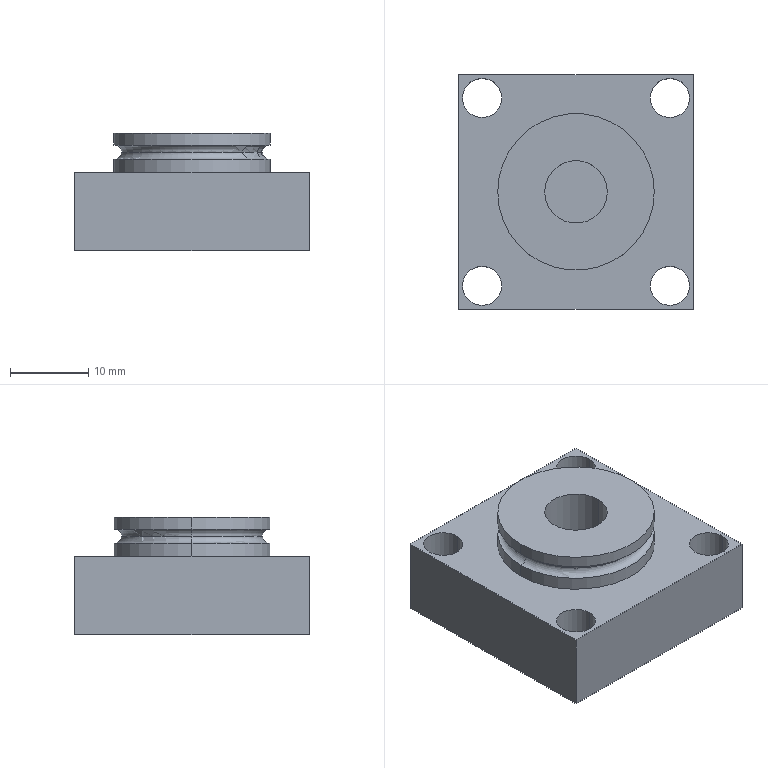Component | SolidWorks | RearEndCapAssembly-1_CylinderRearCover3-1 | 1 solid | 26 faces | box 30 x 30 x 15 mm | volume 9195 mm3 | cylinder 14 | plane 8 | torus 4 | commonest cylinder face diameters 5 x8 20 x4 8 x2
build123d program:
from build123d import *

# Parameters (mm, degrees)
SKETCH1_W         = 30
SKETCH1_H         = 30
EXTRUDE1_DEPTH    = 10
SKETCH2_R         = 10
EXTRUDE2_DEPTH    = 5
SKETCH3_R         = 4
EXTRUDE3_DEPTH    = 10
SKETCH4_R         = 2.5
EXTRUDE4_DEPTH    = 40.125
CIRPATTERN1_COUNT = 4
SKETCH5_R         = 0.9


with BuildPart() as part:
    # Sketch1 → Extrude1 (new body)
    with BuildSketch(Plane.XY):
        with Locations((-19.151, -1.261)):
            Rectangle(SKETCH1_W, SKETCH1_H)
    extrude(amount=EXTRUDE1_DEPTH)

    # Sketch2 → Extrude2 (add)
    with BuildSketch(Plane.XY.offset(10)):
        with Locations((-19.151, -1.261)):
            Circle(SKETCH2_R)
    extrude(amount=EXTRUDE2_DEPTH)

    # Sketch3 → Extrude3 (cut)
    with BuildSketch(Plane.XY.offset(15)):
        with Locations((-19.151, -1.261)):
            Circle(SKETCH3_R)
    extrude(amount=-EXTRUDE3_DEPTH, mode=Mode.SUBTRACT)

    # Sketch4 → Extrude4 (cut, through all)
    with BuildSketch(Plane.XY.offset(10)):
        with Locations((-31.151, 10.739)):
            Circle(SKETCH4_R)
    extrude4 = extrude(amount=-EXTRUDE4_DEPTH, mode=Mode.SUBTRACT)

    # CirPattern1: Extrude4 ×4 about axis
    cirpattern1_axis = Axis((-19.151, -1.261, 0), (0, 0, 1))
    for i in range(1, CIRPATTERN1_COUNT):
        add(extrude4.rotate(cirpattern1_axis, i * 360 / CIRPATTERN1_COUNT), mode=Mode.SUBTRACT)

    # Sketch5 → Cut-Revolve1 (revolve, cut)
    with BuildSketch(Plane(origin=(-19.151, 0, 0), x_dir=(0, 0, -1), z_dir=(1, 0, 0)), mode=Mode.PRIVATE) as cut_revolve1_sk:
        with Locations((-12.6, 8.639)):
            Circle(SKETCH5_R)
    revolve(cut_revolve1_sk.sketch.rotate(Axis((-19.151, -1.261, 5), (0, 0, 1)), 90), axis=Axis((-19.151, -1.261, 5), (0, 0, 1)), mode=Mode.SUBTRACT)


solid = part.part

# Placed as in the assembly
solid = solid.moved(Location((25.276, -0.3856, -7.5), (0, 0, 0)))
STEP:
#1=CARTESIAN_POINT('',(-0.1526,-0.06482,0.1656));
#2=VERTEX_POINT('',#1);
#3=CARTESIAN_POINT('',(-0.1132,-0.06482,0.2008));
#4=VERTEX_POINT('',#3);
#5=CARTESIAN_POINT('',(-0.1486,-0.06482,0.2008));
#6=DIRECTION('',(0.,-1.,0.));
#7=DIRECTION('',(0.,0.,-1.));
#8=AXIS2_PLACEMENT_3D('',#5,#6,#7);
#9=CIRCLE('',#8,0.03543);
#10=EDGE_CURVE('',#2,#4,#9,.T.);
#11=ORIENTED_EDGE('',*,*,#10,.T.);
#12=CARTESIAN_POINT('',(0.5955,-0.06482,0.2008));
#13=VERTEX_POINT('',#12);
#14=CARTESIAN_POINT('',(0.2411,-0.06482,0.2008));
#15=DIRECTION('',(0.,0.,-1.));
#16=DIRECTION('',(-1.,0.,0.));
#17=AXIS2_PLACEMENT_3D('',#14,#15,#16);
#18=CIRCLE('',#17,0.3543);
#19=EDGE_CURVE('',#4,#13,#18,.T.);
#20=ORIENTED_EDGE('',*,*,#19,.T.);
#21=CARTESIAN_POINT('',(0.6348,-0.06482,0.1656));
#22=VERTEX_POINT('',#21);
#23=CARTESIAN_POINT('',(0.6309,-0.06482,0.2008));
#24=DIRECTION('',(-0.,1.,0.));
#25=DIRECTION('',(-1.,-0.,0.));
#26=AXIS2_PLACEMENT_3D('',#23,#24,#25);
#27=CIRCLE('',#26,0.03543);
#28=EDGE_CURVE('',#22,#13,#27,.T.);
#29=ORIENTED_EDGE('',*,*,#28,.F.);
#30=CARTESIAN_POINT('',(0.2411,-0.06482,0.1656));
#31=DIRECTION('',(0.,0.,-1.));
#32=DIRECTION('',(1.,0.,0.));
#33=AXIS2_PLACEMENT_3D('',#30,#31,#32);
#34=CIRCLE('',#33,0.3937);
#35=EDGE_CURVE('',#2,#22,#34,.T.);
#36=ORIENTED_EDGE('',*,*,#35,.F.);
#37=EDGE_LOOP('',(#11,#20,#29,#36));
#38=FACE_OUTER_BOUND('',#37,.T.);
#39=CARTESIAN_POINT('',(0.2411,-0.06482,0.2008));
#40=DIRECTION('',(0.,0.,-1.));
#41=DIRECTION('',(-1.,0.,0.));
#42=AXIS2_PLACEMENT_3D('',#39,#40,#41);
#43=TOROIDAL_SURFACE('',#42,0.3898,0.03543);
#44=ADVANCED_FACE('',(#38),#43,.F.);
#45=ORIENTED_EDGE('',*,*,#28,.T.);
#46=CARTESIAN_POINT('',(0.2411,-0.06482,0.2008));
#47=DIRECTION('',(0.,0.,-1.));
#48=DIRECTION('',(-1.,0.,0.));
#49=AXIS2_PLACEMENT_3D('',#46,#47,#48);
#50=CIRCLE('',#49,0.3543);
#51=EDGE_CURVE('',#13,#4,#50,.T.);
#52=ORIENTED_EDGE('',*,*,#51,.T.);
#53=ORIENTED_EDGE('',*,*,#10,.F.);
#54=CARTESIAN_POINT('',(0.2411,-0.06482,0.1656));
#55=DIRECTION('',(0.,0.,-1.));
#56=DIRECTION('',(1.,0.,0.));
#57=AXIS2_PLACEMENT_3D('',#54,#55,#56);
#58=CIRCLE('',#57,0.3937);
#59=EDGE_CURVE('',#22,#2,#58,.T.);
#60=ORIENTED_EDGE('',*,*,#59,.F.);
#61=EDGE_LOOP('',(#45,#52,#53,#60));
#62=FACE_OUTER_BOUND('',#61,.T.);
#63=CARTESIAN_POINT('',(0.2411,-0.06482,0.2008));
#64=DIRECTION('',(0.,0.,-1.));
#65=DIRECTION('',(-1.,0.,0.));
#66=AXIS2_PLACEMENT_3D('',#63,#64,#65);
#67=TOROIDAL_SURFACE('',#66,0.3898,0.03543);
#68=ADVANCED_FACE('',(#62),#67,.F.);
#69=CARTESIAN_POINT('',(0.6348,-0.06482,0.2953));
#70=VERTEX_POINT('',#69);
#71=CARTESIAN_POINT('',(-0.1526,-0.06482,0.2953));
#72=VERTEX_POINT('',#71);
#73=CARTESIAN_POINT('',(0.2411,-0.06482,0.2953));
#74=DIRECTION('',(0.,0.,1.));
#75=DIRECTION('',(1.,0.,0.));
#76=AXIS2_PLACEMENT_3D('',#73,#74,#75);
#77=CIRCLE('',#76,0.3937);
#78=EDGE_CURVE('',#70,#72,#77,.T.);
#79=ORIENTED_EDGE('',*,*,#78,.F.);
#80=CARTESIAN_POINT('',(0.6348,-0.06482,0.236));
#81=VERTEX_POINT('',#80);
#82=CARTESIAN_POINT('',(0.6348,-0.06482,0.2953));
#83=DIRECTION('',(0.,0.,-1.));
#84=VECTOR('',#83,39.37);
#85=LINE('',#82,#84);
#86=EDGE_CURVE('',#70,#81,#85,.T.);
#87=ORIENTED_EDGE('',*,*,#86,.T.);
#88=CARTESIAN_POINT('',(-0.1526,-0.06482,0.236));
#89=VERTEX_POINT('',#88);
#90=CARTESIAN_POINT('',(0.2411,-0.06482,0.236));
#91=DIRECTION('',(0.,0.,1.));
#92=DIRECTION('',(-1.,0.,0.));
#93=AXIS2_PLACEMENT_3D('',#90,#91,#92);
#94=CIRCLE('',#93,0.3937);
#95=EDGE_CURVE('',#81,#89,#94,.T.);
#96=ORIENTED_EDGE('',*,*,#95,.T.);
#97=CARTESIAN_POINT('',(-0.1526,-0.06482,0.2953));
#98=DIRECTION('',(0.,0.,-1.));
#99=VECTOR('',#98,39.37);
#100=LINE('',#97,#99);
#101=EDGE_CURVE('',#72,#89,#100,.T.);
#102=ORIENTED_EDGE('',*,*,#101,.F.);
#103=EDGE_LOOP('',(#79,#87,#96,#102));
#104=FACE_OUTER_BOUND('',#103,.T.);
#105=CARTESIAN_POINT('',(0.2411,-0.06482,0.2953));
#106=DIRECTION('',(0.,0.,-1.));
#107=DIRECTION('',(-1.,0.,0.));
#108=AXIS2_PLACEMENT_3D('',#105,#106,#107);
#109=CYLINDRICAL_SURFACE('',#108,0.3937);
#110=ADVANCED_FACE('',(#104),#109,.T.);
#111=CARTESIAN_POINT('',(0.08366,-0.06482,-0.09843));
#112=VERTEX_POINT('',#111);
#113=CARTESIAN_POINT('',(0.3986,-0.06482,-0.09843));
#114=VERTEX_POINT('',#113);
#115=CARTESIAN_POINT('',(0.2411,-0.06482,-0.09843));
#116=DIRECTION('',(0.,0.,1.));
#117=DIRECTION('',(1.,0.,0.));
#118=AXIS2_PLACEMENT_3D('',#115,#116,#117);
#119=CIRCLE('',#118,0.1575);
#120=EDGE_CURVE('',#112,#114,#119,.T.);
#121=ORIENTED_EDGE('',*,*,#120,.F.);
#122=CARTESIAN_POINT('',(0.08366,-0.06482,0.2953));
#123=VERTEX_POINT('',#122);
#124=CARTESIAN_POINT('',(0.08366,-0.06482,-0.09843));
#125=DIRECTION('',(0.,0.,1.));
#126=VECTOR('',#125,39.37);
#127=LINE('',#124,#126);
#128=EDGE_CURVE('',#112,#123,#127,.T.);
#129=ORIENTED_EDGE('',*,*,#128,.T.);
#130=CARTESIAN_POINT('',(0.3986,-0.06482,0.2953));
#131=VERTEX_POINT('',#130);
#132=CARTESIAN_POINT('',(0.2411,-0.06482,0.2953));
#133=DIRECTION('',(0.,0.,1.));
#134=DIRECTION('',(1.,0.,0.));
#135=AXIS2_PLACEMENT_3D('',#132,#133,#134);
#136=CIRCLE('',#135,0.1575);
#137=EDGE_CURVE('',#123,#131,#136,.T.);
#138=ORIENTED_EDGE('',*,*,#137,.T.);
#139=CARTESIAN_POINT('',(0.3986,-0.06482,-0.09843));
#140=DIRECTION('',(0.,0.,1.));
#141=VECTOR('',#140,39.37);
#142=LINE('',#139,#141);
#143=EDGE_CURVE('',#114,#131,#142,.T.);
#144=ORIENTED_EDGE('',*,*,#143,.F.);
#145=EDGE_LOOP('',(#121,#129,#138,#144));
#146=FACE_OUTER_BOUND('',#145,.T.);
#147=CARTESIAN_POINT('',(0.2411,-0.06482,-0.09843));
#148=DIRECTION('',(0.,0.,1.));
#149=DIRECTION('',(1.,0.,0.));
#150=AXIS2_PLACEMENT_3D('',#147,#148,#149);
#151=CYLINDRICAL_SURFACE('',#150,0.1575);
#152=ADVANCED_FACE('',(#146),#151,.F.);
#153=ORIENTED_EDGE('',*,*,#51,.F.);
#154=CARTESIAN_POINT('',(0.6309,-0.06482,0.2008));
#155=DIRECTION('',(-0.,1.,0.));
#156=DIRECTION('',(-1.,-0.,0.));
#157=AXIS2_PLACEMENT_3D('',#154,#155,#156);
#158=CIRCLE('',#157,0.03543);
#159=EDGE_CURVE('',#13,#81,#158,.T.);
#160=ORIENTED_EDGE('',*,*,#159,.T.);
#161=CARTESIAN_POINT('',(0.2411,-0.06482,0.236));
#162=DIRECTION('',(0.,0.,1.));
#163=DIRECTION('',(-1.,0.,0.));
#164=AXIS2_PLACEMENT_3D('',#161,#162,#163);
#165=CIRCLE('',#164,0.3937);
#166=EDGE_CURVE('',#89,#81,#165,.T.);
#167=ORIENTED_EDGE('',*,*,#166,.F.);
#168=CARTESIAN_POINT('',(-0.1486,-0.06482,0.2008));
#169=DIRECTION('',(0.,-1.,0.));
#170=DIRECTION('',(0.,0.,-1.));
#171=AXIS2_PLACEMENT_3D('',#168,#169,#170);
#172=CIRCLE('',#171,0.03543);
#173=EDGE_CURVE('',#4,#89,#172,.T.);
#174=ORIENTED_EDGE('',*,*,#173,.F.);
#175=EDGE_LOOP('',(#153,#160,#167,#174));
#176=FACE_OUTER_BOUND('',#175,.T.);
#177=CARTESIAN_POINT('',(0.2411,-0.06482,0.2008));
#178=DIRECTION('',(0.,0.,-1.));
#179=DIRECTION('',(-1.,0.,0.));
#180=AXIS2_PLACEMENT_3D('',#177,#178,#179);
#181=TOROIDAL_SURFACE('',#180,0.3898,0.03543);
#182=ADVANCED_FACE('',(#176),#181,.F.);
#183=CARTESIAN_POINT('',(0.6152,0.4076,-0.2953));
#184=VERTEX_POINT('',#183);
#185=CARTESIAN_POINT('',(0.812,0.4076,-0.2953));
#186=VERTEX_POINT('',#185);
#187=CARTESIAN_POINT('',(0.7136,0.4076,-0.2953));
#188=DIRECTION('',(0.,0.,1.));
#189=DIRECTION('',(0.,-1.,0.));
#190=AXIS2_PLACEMENT_3D('',#187,#188,#189);
#191=CIRCLE('',#190,0.09843);
#192=EDGE_CURVE('',#184,#186,#191,.T.);
#193=ORIENTED_EDGE('',*,*,#192,.F.);
#194=CARTESIAN_POINT('',(0.6152,0.4076,0.09843));
#195=VERTEX_POINT('',#194);
#196=CARTESIAN_POINT('',(0.6152,0.4076,-0.2953));
#197=DIRECTION('',(0.,0.,1.));
#198=VECTOR('',#197,39.37);
#199=LINE('',#196,#198);
#200=EDGE_CURVE('',#184,#195,#199,.T.);
#201=ORIENTED_EDGE('',*,*,#200,.T.);
#202=CARTESIAN_POINT('',(0.812,0.4076,0.09843));
#203=VERTEX_POINT('',#202);
#204=CARTESIAN_POINT('',(0.7136,0.4076,0.09843));
#205=DIRECTION('',(0.,0.,1.));
#206=DIRECTION('',(0.,-1.,0.));
#207=AXIS2_PLACEMENT_3D('',#204,#205,#206);
#208=CIRCLE('',#207,0.09843);
#209=EDGE_CURVE('',#195,#203,#208,.T.);
#210=ORIENTED_EDGE('',*,*,#209,.T.);
#211=CARTESIAN_POINT('',(0.812,0.4076,-0.2953));
#212=DIRECTION('',(0.,0.,1.));
#213=VECTOR('',#212,39.37);
#214=LINE('',#211,#213);
#215=EDGE_CURVE('',#186,#203,#214,.T.);
#216=ORIENTED_EDGE('',*,*,#215,.F.);
#217=EDGE_LOOP('',(#193,#201,#210,#216));
#218=FACE_OUTER_BOUND('',#217,.T.);
#219=CARTESIAN_POINT('',(0.7136,0.4076,-0.2953));
#220=DIRECTION('',(0.,0.,1.));
#221=DIRECTION('',(1.,0.,0.));
#222=AXIS2_PLACEMENT_3D('',#219,#220,#221);
#223=CYLINDRICAL_SURFACE('',#222,0.09843);
#224=ADVANCED_FACE('',(#218),#223,.F.);
#225=CARTESIAN_POINT('',(0.6152,-0.5373,-0.2953));
#226=VERTEX_POINT('',#225);
#227=CARTESIAN_POINT('',(0.812,-0.5373,-0.2953));
#228=VERTEX_POINT('',#227);
#229=CARTESIAN_POINT('',(0.7136,-0.5373,-0.2953));
#230=DIRECTION('',(0.,0.,1.));
#231=DIRECTION('',(-1.,-0.,0.));
#232=AXIS2_PLACEMENT_3D('',#229,#230,#231);
#233=CIRCLE('',#232,0.09843);
#234=EDGE_CURVE('',#226,#228,#233,.T.);
#235=ORIENTED_EDGE('',*,*,#234,.F.);
#236=CARTESIAN_POINT('',(0.6152,-0.5373,0.09843));
#237=VERTEX_POINT('',#236);
#238=CARTESIAN_POINT('',(0.6152,-0.5373,-0.2953));
#239=DIRECTION('',(0.,0.,1.));
#240=VECTOR('',#239,39.37);
#241=LINE('',#238,#240);
#242=EDGE_CURVE('',#226,#237,#241,.T.);
#243=ORIENTED_EDGE('',*,*,#242,.T.);
#244=CARTESIAN_POINT('',(0.812,-0.5373,0.09843));
#245=VERTEX_POINT('',#244);
#246=CARTESIAN_POINT('',(0.7136,-0.5373,0.09843));
#247=DIRECTION('',(0.,0.,1.));
#248=DIRECTION('',(-1.,-0.,0.));
#249=AXIS2_PLACEMENT_3D('',#246,#247,#248);
#250=CIRCLE('',#249,0.09843);
#251=EDGE_CURVE('',#237,#245,#250,.T.);
#252=ORIENTED_EDGE('',*,*,#251,.T.);
#253=CARTESIAN_POINT('',(0.812,-0.5373,-0.2953));
#254=DIRECTION('',(0.,0.,1.));
#255=VECTOR('',#254,39.37);
#256=LINE('',#253,#255);
#257=EDGE_CURVE('',#228,#245,#256,.T.);
#258=ORIENTED_EDGE('',*,*,#257,.F.);
#259=EDGE_LOOP('',(#235,#243,#252,#258));
#260=FACE_OUTER_BOUND('',#259,.T.);
#261=CARTESIAN_POINT('',(0.7136,-0.5373,-0.2953));
#262=DIRECTION('',(0.,0.,1.));
#263=DIRECTION('',(1.,0.,0.));
#264=AXIS2_PLACEMENT_3D('',#261,#262,#263);
#265=CYLINDRICAL_SURFACE('',#264,0.09843);
#266=ADVANCED_FACE('',(#260),#265,.F.);
#267=CARTESIAN_POINT('',(-0.3297,-0.5373,-0.2953));
#268=VERTEX_POINT('',#267);
#269=CARTESIAN_POINT('',(-0.1329,-0.5373,-0.2953));
#270=VERTEX_POINT('',#269);
#271=CARTESIAN_POINT('',(-0.2313,-0.5373,-0.2953));
#272=DIRECTION('',(0.,0.,1.));
#273=DIRECTION('',(-0.,1.,0.));
#274=AXIS2_PLACEMENT_3D('',#271,#272,#273);
#275=CIRCLE('',#274,0.09843);
#276=EDGE_CURVE('',#268,#270,#275,.T.);
#277=ORIENTED_EDGE('',*,*,#276,.F.);
#278=CARTESIAN_POINT('',(-0.3297,-0.5373,0.09843));
#279=VERTEX_POINT('',#278);
#280=CARTESIAN_POINT('',(-0.3297,-0.5373,-0.2953));
#281=DIRECTION('',(0.,0.,1.));
#282=VECTOR('',#281,39.37);
#283=LINE('',#280,#282);
#284=EDGE_CURVE('',#268,#279,#283,.T.);
#285=ORIENTED_EDGE('',*,*,#284,.T.);
#286=CARTESIAN_POINT('',(-0.1329,-0.5373,0.09843));
#287=VERTEX_POINT('',#286);
#288=CARTESIAN_POINT('',(-0.2313,-0.5373,0.09843));
#289=DIRECTION('',(0.,0.,1.));
#290=DIRECTION('',(-0.,1.,0.));
#291=AXIS2_PLACEMENT_3D('',#288,#289,#290);
#292=CIRCLE('',#291,0.09843);
#293=EDGE_CURVE('',#279,#287,#292,.T.);
#294=ORIENTED_EDGE('',*,*,#293,.T.);
#295=CARTESIAN_POINT('',(-0.1329,-0.5373,-0.2953));
#296=DIRECTION('',(0.,0.,1.));
#297=VECTOR('',#296,39.37);
#298=LINE('',#295,#297);
#299=EDGE_CURVE('',#270,#287,#298,.T.);
#300=ORIENTED_EDGE('',*,*,#299,.F.);
#301=EDGE_LOOP('',(#277,#285,#294,#300));
#302=FACE_OUTER_BOUND('',#301,.T.);
#303=CARTESIAN_POINT('',(-0.2313,-0.5373,-0.2953));
#304=DIRECTION('',(0.,0.,1.));
#305=DIRECTION('',(1.,0.,0.));
#306=AXIS2_PLACEMENT_3D('',#303,#304,#305);
#307=CYLINDRICAL_SURFACE('',#306,0.09843);
#308=ADVANCED_FACE('',(#302),#307,.F.);
#309=CARTESIAN_POINT('',(-0.3297,0.4076,-0.2953));
#310=VERTEX_POINT('',#309);
#311=CARTESIAN_POINT('',(-0.1329,0.4076,-0.2953));
#312=VERTEX_POINT('',#311);
#313=CARTESIAN_POINT('',(-0.2313,0.4076,-0.2953));
#314=DIRECTION('',(0.,0.,1.));
#315=DIRECTION('',(1.,0.,0.));
#316=AXIS2_PLACEMENT_3D('',#313,#314,#315);
#317=CIRCLE('',#316,0.09843);
#318=EDGE_CURVE('',#310,#312,#317,.T.);
#319=ORIENTED_EDGE('',*,*,#318,.F.);
#320=CARTESIAN_POINT('',(-0.3297,0.4076,0.09843));
#321=VERTEX_POINT('',#320);
#322=CARTESIAN_POINT('',(-0.3297,0.4076,-0.2953));
#323=DIRECTION('',(0.,0.,1.));
#324=VECTOR('',#323,39.37);
#325=LINE('',#322,#324);
#326=EDGE_CURVE('',#310,#321,#325,.T.);
#327=ORIENTED_EDGE('',*,*,#326,.T.);
#328=CARTESIAN_POINT('',(-0.1329,0.4076,0.09843));
#329=VERTEX_POINT('',#328);
#330=CARTESIAN_POINT('',(-0.2313,0.4076,0.09843));
#331=DIRECTION('',(0.,0.,1.));
#332=DIRECTION('',(1.,0.,0.));
#333=AXIS2_PLACEMENT_3D('',#330,#331,#332);
#334=CIRCLE('',#333,0.09843);
#335=EDGE_CURVE('',#321,#329,#334,.T.);
#336=ORIENTED_EDGE('',*,*,#335,.T.);
#337=CARTESIAN_POINT('',(-0.1329,0.4076,-0.2953));
#338=DIRECTION('',(0.,0.,1.));
#339=VECTOR('',#338,39.37);
#340=LINE('',#337,#339);
#341=EDGE_CURVE('',#312,#329,#340,.T.);
#342=ORIENTED_EDGE('',*,*,#341,.F.);
#343=EDGE_LOOP('',(#319,#327,#336,#342));
#344=FACE_OUTER_BOUND('',#343,.T.);
#345=CARTESIAN_POINT('',(-0.2313,0.4076,-0.2953));
#346=DIRECTION('',(0.,0.,1.));
#347=DIRECTION('',(1.,0.,0.));
#348=AXIS2_PLACEMENT_3D('',#345,#346,#347);
#349=CYLINDRICAL_SURFACE('',#348,0.09843);
#350=ADVANCED_FACE('',(#344),#349,.F.);
#351=ORIENTED_EDGE('',*,*,#35,.T.);
#352=CARTESIAN_POINT('',(0.6348,-0.06482,0.09843));
#353=VERTEX_POINT('',#352);
#354=CARTESIAN_POINT('',(0.6348,-0.06482,0.2953));
#355=DIRECTION('',(0.,0.,-1.));
#356=VECTOR('',#355,39.37);
#357=LINE('',#354,#356);
#358=EDGE_CURVE('',#22,#353,#357,.T.);
#359=ORIENTED_EDGE('',*,*,#358,.T.);
#360=CARTESIAN_POINT('',(-0.1526,-0.06482,0.09843));
#361=VERTEX_POINT('',#360);
#362=CARTESIAN_POINT('',(0.2411,-0.06482,0.09843));
#363=DIRECTION('',(0.,0.,1.));
#364=DIRECTION('',(1.,0.,0.));
#365=AXIS2_PLACEMENT_3D('',#362,#363,#364);
#366=CIRCLE('',#365,0.3937);
#367=EDGE_CURVE('',#353,#361,#366,.T.);
#368=ORIENTED_EDGE('',*,*,#367,.T.);
#369=CARTESIAN_POINT('',(-0.1526,-0.06482,0.2953));
#370=DIRECTION('',(0.,0.,-1.));
#371=VECTOR('',#370,39.37);
#372=LINE('',#369,#371);
#373=EDGE_CURVE('',#2,#361,#372,.T.);
#374=ORIENTED_EDGE('',*,*,#373,.F.);
#375=EDGE_LOOP('',(#351,#359,#368,#374));
#376=FACE_OUTER_BOUND('',#375,.T.);
#377=CARTESIAN_POINT('',(0.2411,-0.06482,0.2953));
#378=DIRECTION('',(0.,0.,-1.));
#379=DIRECTION('',(-1.,0.,0.));
#380=AXIS2_PLACEMENT_3D('',#377,#378,#379);
#381=CYLINDRICAL_SURFACE('',#380,0.3937);
#382=ADVANCED_FACE('',(#376),#381,.T.);
#383=ORIENTED_EDGE('',*,*,#358,.F.);
#384=ORIENTED_EDGE('',*,*,#59,.T.);
#385=ORIENTED_EDGE('',*,*,#373,.T.);
#386=CARTESIAN_POINT('',(0.2411,-0.06482,0.09843));
#387=DIRECTION('',(0.,0.,1.));
#388=DIRECTION('',(1.,0.,0.));
#389=AXIS2_PLACEMENT_3D('',#386,#387,#388);
#390=CIRCLE('',#389,0.3937);
#391=EDGE_CURVE('',#361,#353,#390,.T.);
#392=ORIENTED_EDGE('',*,*,#391,.T.);
#393=EDGE_LOOP('',(#383,#384,#385,#392));
#394=FACE_OUTER_BOUND('',#393,.T.);
#395=CARTESIAN_POINT('',(0.2411,-0.06482,0.2953));
#396=DIRECTION('',(0.,0.,-1.));
#397=DIRECTION('',(-1.,0.,0.));
#398=AXIS2_PLACEMENT_3D('',#395,#396,#397);
#399=CYLINDRICAL_SURFACE('',#398,0.3937);
#400=ADVANCED_FACE('',(#394),#399,.T.);
#401=CARTESIAN_POINT('',(0.7136,0.4076,0.09843));
#402=DIRECTION('',(0.,0.,1.));
#403=DIRECTION('',(0.,-1.,0.));
#404=AXIS2_PLACEMENT_3D('',#401,#402,#403);
#405=CIRCLE('',#404,0.09843);
#406=EDGE_CURVE('',#203,#195,#405,.T.);
#407=ORIENTED_EDGE('',*,*,#406,.F.);
#408=ORIENTED_EDGE('',*,*,#209,.F.);
#409=EDGE_LOOP('',(#407,#408));
#410=FACE_BOUND('',#409,.T.);
#411=CARTESIAN_POINT('',(0.7136,-0.5373,0.09843));
#412=DIRECTION('',(0.,0.,1.));
#413=DIRECTION('',(-1.,-0.,0.));
#414=AXIS2_PLACEMENT_3D('',#411,#412,#413);
#415=CIRCLE('',#414,0.09843);
#416=EDGE_CURVE('',#245,#237,#415,.T.);
#417=ORIENTED_EDGE('',*,*,#416,.F.);
#418=ORIENTED_EDGE('',*,*,#251,.F.);
#419=EDGE_LOOP('',(#417,#418));
#420=FACE_BOUND('',#419,.T.);
#421=CARTESIAN_POINT('',(-0.2313,-0.5373,0.09843));
#422=DIRECTION('',(0.,0.,1.));
#423=DIRECTION('',(-0.,1.,0.));
#424=AXIS2_PLACEMENT_3D('',#421,#422,#423);
#425=CIRCLE('',#424,0.09843);
#426=EDGE_CURVE('',#287,#279,#425,.T.);
#427=ORIENTED_EDGE('',*,*,#426,.F.);
#428=ORIENTED_EDGE('',*,*,#293,.F.);
#429=EDGE_LOOP('',(#427,#428));
#430=FACE_BOUND('',#429,.T.);
#431=CARTESIAN_POINT('',(-0.2313,0.4076,0.09843));
#432=DIRECTION('',(0.,0.,1.));
#433=DIRECTION('',(1.,0.,0.));
#434=AXIS2_PLACEMENT_3D('',#431,#432,#433);
#435=CIRCLE('',#434,0.09843);
#436=EDGE_CURVE('',#329,#321,#435,.T.);
#437=ORIENTED_EDGE('',*,*,#436,.F.);
#438=ORIENTED_EDGE('',*,*,#335,.F.);
#439=EDGE_LOOP('',(#437,#438));
#440=FACE_BOUND('',#439,.T.);
#441=CARTESIAN_POINT('',(-0.3494,0.5257,0.09843));
#442=VERTEX_POINT('',#441);
#443=CARTESIAN_POINT('',(-0.3494,-0.6554,0.09843));
#444=VERTEX_POINT('',#443);
#445=CARTESIAN_POINT('',(-0.3494,0.5257,0.09843));
#446=DIRECTION('',(0.,-1.,0.));
#447=VECTOR('',#446,39.37);
#448=LINE('',#445,#447);
#449=EDGE_CURVE('',#442,#444,#448,.T.);
#450=ORIENTED_EDGE('',*,*,#449,.T.);
#451=CARTESIAN_POINT('',(0.8317,-0.6554,0.09843));
#452=VERTEX_POINT('',#451);
#453=CARTESIAN_POINT('',(-0.3494,-0.6554,0.09843));
#454=DIRECTION('',(1.,0.,0.));
#455=VECTOR('',#454,39.37);
#456=LINE('',#453,#455);
#457=EDGE_CURVE('',#444,#452,#456,.T.);
#458=ORIENTED_EDGE('',*,*,#457,.T.);
#459=CARTESIAN_POINT('',(0.8317,0.5257,0.09843));
#460=VERTEX_POINT('',#459);
#461=CARTESIAN_POINT('',(0.8317,0.5257,0.09843));
#462=DIRECTION('',(-0.,1.,0.));
#463=VECTOR('',#462,39.37);
#464=LINE('',#461,#463);
#465=EDGE_CURVE('',#452,#460,#464,.T.);
#466=ORIENTED_EDGE('',*,*,#465,.T.);
#467=CARTESIAN_POINT('',(-0.3494,0.5257,0.09843));
#468=DIRECTION('',(-1.,0.,0.));
#469=VECTOR('',#468,39.37);
#470=LINE('',#467,#469);
#471=EDGE_CURVE('',#460,#442,#470,.T.);
#472=ORIENTED_EDGE('',*,*,#471,.T.);
#473=EDGE_LOOP('',(#450,#458,#466,#472));
#474=FACE_OUTER_BOUND('',#473,.T.);
#475=ORIENTED_EDGE('',*,*,#391,.F.);
#476=ORIENTED_EDGE('',*,*,#367,.F.);
#477=EDGE_LOOP('',(#475,#476));
#478=FACE_BOUND('',#477,.T.);
#479=CARTESIAN_POINT('',(-0.3494,-0.6554,0.09843));
#480=DIRECTION('',(0.,0.,1.));
#481=DIRECTION('',(1.,0.,0.));
#482=AXIS2_PLACEMENT_3D('',#479,#480,#481);
#483=PLANE('',#482);
#484=ADVANCED_FACE('',(#410,#420,#430,#440,#474,#478),#483,.T.);
#485=CARTESIAN_POINT('',(-0.3494,0.5257,-0.2953));
#486=VERTEX_POINT('',#485);
#487=CARTESIAN_POINT('',(-0.3494,-0.6554,-0.2953));
#488=VERTEX_POINT('',#487);
#489=CARTESIAN_POINT('',(-0.3494,0.5257,-0.2953));
#490=DIRECTION('',(0.,-1.,0.));
#491=VECTOR('',#490,39.37);
#492=LINE('',#489,#491);
#493=EDGE_CURVE('',#486,#488,#492,.T.);
#494=ORIENTED_EDGE('',*,*,#493,.T.);
#495=CARTESIAN_POINT('',(-0.3494,-0.6554,0.09843));
#496=DIRECTION('',(0.,0.,-1.));
#497=VECTOR('',#496,39.37);
#498=LINE('',#495,#497);
#499=EDGE_CURVE('',#444,#488,#498,.T.);
#500=ORIENTED_EDGE('',*,*,#499,.F.);
#501=ORIENTED_EDGE('',*,*,#449,.F.);
#502=CARTESIAN_POINT('',(-0.3494,0.5257,0.09843));
#503=DIRECTION('',(0.,0.,-1.));
#504=VECTOR('',#503,39.37);
#505=LINE('',#502,#504);
#506=EDGE_CURVE('',#442,#486,#505,.T.);
#507=ORIENTED_EDGE('',*,*,#506,.T.);
#508=EDGE_LOOP('',(#494,#500,#501,#507));
#509=FACE_OUTER_BOUND('',#508,.T.);
#510=CARTESIAN_POINT('',(-0.3494,0.5257,0.09843));
#511=DIRECTION('',(1.,0.,0.));
#512=DIRECTION('',(-0.,1.,0.));
#513=AXIS2_PLACEMENT_3D('',#510,#511,#512);
#514=PLANE('',#513);
#515=ADVANCED_FACE('',(#509),#514,.F.);
#516=CARTESIAN_POINT('',(0.8317,-0.6554,-0.2953));
#517=VERTEX_POINT('',#516);
#518=CARTESIAN_POINT('',(-0.3494,-0.6554,-0.2953));
#519=DIRECTION('',(1.,0.,0.));
#520=VECTOR('',#519,39.37);
#521=LINE('',#518,#520);
#522=EDGE_CURVE('',#488,#517,#521,.T.);
#523=ORIENTED_EDGE('',*,*,#522,.T.);
#524=CARTESIAN_POINT('',(0.8317,-0.6554,0.09843));
#525=DIRECTION('',(0.,0.,-1.));
#526=VECTOR('',#525,39.37);
#527=LINE('',#524,#526);
#528=EDGE_CURVE('',#452,#517,#527,.T.);
#529=ORIENTED_EDGE('',*,*,#528,.F.);
#530=ORIENTED_EDGE('',*,*,#457,.F.);
#531=ORIENTED_EDGE('',*,*,#499,.T.);
#532=EDGE_LOOP('',(#523,#529,#530,#531));
#533=FACE_OUTER_BOUND('',#532,.T.);
#534=CARTESIAN_POINT('',(-0.3494,-0.6554,0.09843));
#535=DIRECTION('',(0.,1.,0.));
#536=DIRECTION('',(0.,0.,1.));
#537=AXIS2_PLACEMENT_3D('',#534,#535,#536);
#538=PLANE('',#537);
#539=ADVANCED_FACE('',(#533),#538,.F.);
#540=CARTESIAN_POINT('',(0.8317,0.5257,-0.2953));
#541=VERTEX_POINT('',#540);
#542=CARTESIAN_POINT('',(0.8317,0.5257,-0.2953));
#543=DIRECTION('',(-0.,1.,0.));
#544=VECTOR('',#543,39.37);
#545=LINE('',#542,#544);
#546=EDGE_CURVE('',#517,#541,#545,.T.);
#547=ORIENTED_EDGE('',*,*,#546,.T.);
#548=CARTESIAN_POINT('',(0.8317,0.5257,0.09843));
#549=DIRECTION('',(0.,0.,-1.));
#550=VECTOR('',#549,39.37);
#551=LINE('',#548,#550);
#552=EDGE_CURVE('',#460,#541,#551,.T.);
#553=ORIENTED_EDGE('',*,*,#552,.F.);
#554=ORIENTED_EDGE('',*,*,#465,.F.);
#555=ORIENTED_EDGE('',*,*,#528,.T.);
#556=EDGE_LOOP('',(#547,#553,#554,#555));
#557=FACE_OUTER_BOUND('',#556,.T.);
#558=CARTESIAN_POINT('',(0.8317,0.5257,0.09843));
#559=DIRECTION('',(-1.,-0.,0.));
#560=DIRECTION('',(0.,-1.,0.));
#561=AXIS2_PLACEMENT_3D('',#558,#559,#560);
#562=PLANE('',#561);
#563=ADVANCED_FACE('',(#557),#562,.F.);
#564=CARTESIAN_POINT('',(-0.3494,0.5257,-0.2953));
#565=DIRECTION('',(-1.,0.,0.));
#566=VECTOR('',#565,39.37);
#567=LINE('',#564,#566);
#568=EDGE_CURVE('',#541,#486,#567,.T.);
#569=ORIENTED_EDGE('',*,*,#568,.T.);
#570=ORIENTED_EDGE('',*,*,#506,.F.);
#571=ORIENTED_EDGE('',*,*,#471,.F.);
#572=ORIENTED_EDGE('',*,*,#552,.T.);
#573=EDGE_LOOP('',(#569,#570,#571,#572));
#574=FACE_OUTER_BOUND('',#573,.T.);
#575=CARTESIAN_POINT('',(-0.3494,0.5257,0.09843));
#576=DIRECTION('',(0.,-1.,0.));
#577=DIRECTION('',(0.,0.,-1.));
#578=AXIS2_PLACEMENT_3D('',#575,#576,#577);
#579=PLANE('',#578);
#580=ADVANCED_FACE('',(#574),#579,.F.);
#581=CARTESIAN_POINT('',(0.7136,0.4076,-0.2953));
#582=DIRECTION('',(0.,0.,1.));
#583=DIRECTION('',(0.,-1.,0.));
#584=AXIS2_PLACEMENT_3D('',#581,#582,#583);
#585=CIRCLE('',#584,0.09843);
#586=EDGE_CURVE('',#186,#184,#585,.T.);
#587=ORIENTED_EDGE('',*,*,#586,.T.);
#588=ORIENTED_EDGE('',*,*,#192,.T.);
#589=EDGE_LOOP('',(#587,#588));
#590=FACE_BOUND('',#589,.T.);
#591=CARTESIAN_POINT('',(0.7136,-0.5373,-0.2953));
#592=DIRECTION('',(0.,0.,1.));
#593=DIRECTION('',(-1.,-0.,0.));
#594=AXIS2_PLACEMENT_3D('',#591,#592,#593);
#595=CIRCLE('',#594,0.09843);
#596=EDGE_CURVE('',#228,#226,#595,.T.);
#597=ORIENTED_EDGE('',*,*,#596,.T.);
#598=ORIENTED_EDGE('',*,*,#234,.T.);
#599=EDGE_LOOP('',(#597,#598));
#600=FACE_BOUND('',#599,.T.);
#601=CARTESIAN_POINT('',(-0.2313,-0.5373,-0.2953));
#602=DIRECTION('',(0.,0.,1.));
#603=DIRECTION('',(-0.,1.,0.));
#604=AXIS2_PLACEMENT_3D('',#601,#602,#603);
#605=CIRCLE('',#604,0.09843);
#606=EDGE_CURVE('',#270,#268,#605,.T.);
#607=ORIENTED_EDGE('',*,*,#606,.T.);
#608=ORIENTED_EDGE('',*,*,#276,.T.);
#609=EDGE_LOOP('',(#607,#608));
#610=FACE_BOUND('',#609,.T.);
#611=CARTESIAN_POINT('',(-0.2313,0.4076,-0.2953));
#612=DIRECTION('',(0.,0.,1.));
#613=DIRECTION('',(1.,0.,0.));
#614=AXIS2_PLACEMENT_3D('',#611,#612,#613);
#615=CIRCLE('',#614,0.09843);
#616=EDGE_CURVE('',#312,#310,#615,.T.);
#617=ORIENTED_EDGE('',*,*,#616,.T.);
#618=ORIENTED_EDGE('',*,*,#318,.T.);
#619=EDGE_LOOP('',(#617,#618));
#620=FACE_BOUND('',#619,.T.);
#621=ORIENTED_EDGE('',*,*,#493,.F.);
#622=ORIENTED_EDGE('',*,*,#568,.F.);
#623=ORIENTED_EDGE('',*,*,#546,.F.);
#624=ORIENTED_EDGE('',*,*,#522,.F.);
#625=EDGE_LOOP('',(#621,#622,#623,#624));
#626=FACE_OUTER_BOUND('',#625,.T.);
#627=CARTESIAN_POINT('',(-0.3494,-0.6554,-0.2953));
#628=DIRECTION('',(0.,0.,1.));
#629=DIRECTION('',(1.,0.,0.));
#630=AXIS2_PLACEMENT_3D('',#627,#628,#629);
#631=PLANE('',#630);
#632=ADVANCED_FACE('',(#590,#600,#610,#620,#626),#631,.F.);
#633=ORIENTED_EDGE('',*,*,#326,.F.);
#634=ORIENTED_EDGE('',*,*,#616,.F.);
#635=ORIENTED_EDGE('',*,*,#341,.T.);
#636=ORIENTED_EDGE('',*,*,#436,.T.);
#637=EDGE_LOOP('',(#633,#634,#635,#636));
#638=FACE_OUTER_BOUND('',#637,.T.);
#639=CARTESIAN_POINT('',(-0.2313,0.4076,-0.2953));
#640=DIRECTION('',(0.,0.,1.));
#641=DIRECTION('',(1.,0.,0.));
#642=AXIS2_PLACEMENT_3D('',#639,#640,#641);
#643=CYLINDRICAL_SURFACE('',#642,0.09843);
#644=ADVANCED_FACE('',(#638),#643,.F.);
#645=ORIENTED_EDGE('',*,*,#284,.F.);
#646=ORIENTED_EDGE('',*,*,#606,.F.);
#647=ORIENTED_EDGE('',*,*,#299,.T.);
#648=ORIENTED_EDGE('',*,*,#426,.T.);
#649=EDGE_LOOP('',(#645,#646,#647,#648));
#650=FACE_OUTER_BOUND('',#649,.T.);
#651=CARTESIAN_POINT('',(-0.2313,-0.5373,-0.2953));
#652=DIRECTION('',(0.,0.,1.));
#653=DIRECTION('',(1.,0.,0.));
#654=AXIS2_PLACEMENT_3D('',#651,#652,#653);
#655=CYLINDRICAL_SURFACE('',#654,0.09843);
#656=ADVANCED_FACE('',(#650),#655,.F.);
#657=ORIENTED_EDGE('',*,*,#242,.F.);
#658=ORIENTED_EDGE('',*,*,#596,.F.);
#659=ORIENTED_EDGE('',*,*,#257,.T.);
#660=ORIENTED_EDGE('',*,*,#416,.T.);
#661=EDGE_LOOP('',(#657,#658,#659,#660));
#662=FACE_OUTER_BOUND('',#661,.T.);
#663=CARTESIAN_POINT('',(0.7136,-0.5373,-0.2953));
#664=DIRECTION('',(0.,0.,1.));
#665=DIRECTION('',(1.,0.,0.));
#666=AXIS2_PLACEMENT_3D('',#663,#664,#665);
#667=CYLINDRICAL_SURFACE('',#666,0.09843);
#668=ADVANCED_FACE('',(#662),#667,.F.);
#669=ORIENTED_EDGE('',*,*,#200,.F.);
#670=ORIENTED_EDGE('',*,*,#586,.F.);
#671=ORIENTED_EDGE('',*,*,#215,.T.);
#672=ORIENTED_EDGE('',*,*,#406,.T.);
#673=EDGE_LOOP('',(#669,#670,#671,#672));
#674=FACE_OUTER_BOUND('',#673,.T.);
#675=CARTESIAN_POINT('',(0.7136,0.4076,-0.2953));
#676=DIRECTION('',(0.,0.,1.));
#677=DIRECTION('',(1.,0.,0.));
#678=AXIS2_PLACEMENT_3D('',#675,#676,#677);
#679=CYLINDRICAL_SURFACE('',#678,0.09843);
#680=ADVANCED_FACE('',(#674),#679,.F.);
#681=ORIENTED_EDGE('',*,*,#19,.F.);
#682=ORIENTED_EDGE('',*,*,#173,.T.);
#683=ORIENTED_EDGE('',*,*,#95,.F.);
#684=ORIENTED_EDGE('',*,*,#159,.F.);
#685=EDGE_LOOP('',(#681,#682,#683,#684));
#686=FACE_OUTER_BOUND('',#685,.T.);
#687=CARTESIAN_POINT('',(0.2411,-0.06482,0.2008));
#688=DIRECTION('',(0.,0.,-1.));
#689=DIRECTION('',(-1.,0.,0.));
#690=AXIS2_PLACEMENT_3D('',#687,#688,#689);
#691=TOROIDAL_SURFACE('',#690,0.3898,0.03543);
#692=ADVANCED_FACE('',(#686),#691,.F.);
#693=CARTESIAN_POINT('',(0.2411,-0.06482,-0.09843));
#694=DIRECTION('',(0.,0.,1.));
#695=DIRECTION('',(1.,0.,0.));
#696=AXIS2_PLACEMENT_3D('',#693,#694,#695);
#697=CIRCLE('',#696,0.1575);
#698=EDGE_CURVE('',#114,#112,#697,.T.);
#699=ORIENTED_EDGE('',*,*,#698,.T.);
#700=ORIENTED_EDGE('',*,*,#120,.T.);
#701=EDGE_LOOP('',(#699,#700));
#702=FACE_OUTER_BOUND('',#701,.T.);
#703=CARTESIAN_POINT('',(0.2411,-0.06482,-0.09843));
#704=DIRECTION('',(0.,0.,1.));
#705=DIRECTION('',(1.,0.,0.));
#706=AXIS2_PLACEMENT_3D('',#703,#704,#705);
#707=PLANE('',#706);
#708=ADVANCED_FACE('',(#702),#707,.T.);
#709=ORIENTED_EDGE('',*,*,#128,.F.);
#710=ORIENTED_EDGE('',*,*,#698,.F.);
#711=ORIENTED_EDGE('',*,*,#143,.T.);
#712=CARTESIAN_POINT('',(0.2411,-0.06482,0.2953));
#713=DIRECTION('',(0.,0.,1.));
#714=DIRECTION('',(1.,0.,0.));
#715=AXIS2_PLACEMENT_3D('',#712,#713,#714);
#716=CIRCLE('',#715,0.1575);
#717=EDGE_CURVE('',#131,#123,#716,.T.);
#718=ORIENTED_EDGE('',*,*,#717,.T.);
#719=EDGE_LOOP('',(#709,#710,#711,#718));
#720=FACE_OUTER_BOUND('',#719,.T.);
#721=CARTESIAN_POINT('',(0.2411,-0.06482,-0.09843));
#722=DIRECTION('',(0.,0.,1.));
#723=DIRECTION('',(1.,0.,0.));
#724=AXIS2_PLACEMENT_3D('',#721,#722,#723);
#725=CYLINDRICAL_SURFACE('',#724,0.1575);
#726=ADVANCED_FACE('',(#720),#725,.F.);
#727=ORIENTED_EDGE('',*,*,#717,.F.);
#728=ORIENTED_EDGE('',*,*,#137,.F.);
#729=EDGE_LOOP('',(#727,#728));
#730=FACE_BOUND('',#729,.T.);
#731=CARTESIAN_POINT('',(0.2411,-0.06482,0.2953));
#732=DIRECTION('',(0.,0.,1.));
#733=DIRECTION('',(1.,0.,0.));
#734=AXIS2_PLACEMENT_3D('',#731,#732,#733);
#735=CIRCLE('',#734,0.3937);
#736=EDGE_CURVE('',#72,#70,#735,.T.);
#737=ORIENTED_EDGE('',*,*,#736,.T.);
#738=ORIENTED_EDGE('',*,*,#78,.T.);
#739=EDGE_LOOP('',(#737,#738));
#740=FACE_OUTER_BOUND('',#739,.T.);
#741=CARTESIAN_POINT('',(0.2411,-0.06482,0.2953));
#742=DIRECTION('',(0.,0.,1.));
#743=DIRECTION('',(1.,0.,0.));
#744=AXIS2_PLACEMENT_3D('',#741,#742,#743);
#745=PLANE('',#744);
#746=ADVANCED_FACE('',(#730,#740),#745,.T.);
#747=ORIENTED_EDGE('',*,*,#86,.F.);
#748=ORIENTED_EDGE('',*,*,#736,.F.);
#749=ORIENTED_EDGE('',*,*,#101,.T.);
#750=ORIENTED_EDGE('',*,*,#166,.T.);
#751=EDGE_LOOP('',(#747,#748,#749,#750));
#752=FACE_OUTER_BOUND('',#751,.T.);
#753=CARTESIAN_POINT('',(0.2411,-0.06482,0.2953));
#754=DIRECTION('',(0.,0.,-1.));
#755=DIRECTION('',(-1.,0.,0.));
#756=AXIS2_PLACEMENT_3D('',#753,#754,#755);
#757=CYLINDRICAL_SURFACE('',#756,0.3937);
#758=ADVANCED_FACE('',(#752),#757,.T.);
#759=CLOSED_SHELL('',(#44,#68,#110,#152,#182,#224,#266,#308,#350,#382,#400,#484,#515,#539,#563,#580,#632,#644,#656,#668,#680,#692,#708,#726,#746,#758));
#760=MANIFOLD_SOLID_BREP('',#759);
#761=CARTESIAN_POINT('',(0.,0.,0.));
#762=DIRECTION('',(0.,0.,1.));
#763=DIRECTION('',(1.,0.,0.));
#764=AXIS2_PLACEMENT_3D('',#761,#762,#763);
#765=(LENGTH_UNIT()NAMED_UNIT(*)SI_UNIT($,.METRE.));
#766=LENGTH_MEASURE_WITH_UNIT(LENGTH_MEASURE(0.0254),#765);
#767=DIMENSIONAL_EXPONENTS(1.,0.,0.,0.,0.,0.,0.);
#768=(CONVERSION_BASED_UNIT('',#766)LENGTH_UNIT()NAMED_UNIT(#767));
#769=UNCERTAINTY_MEASURE_WITH_UNIT(LENGTH_MEASURE(0.00001),#768,'','');
#770=(NAMED_UNIT(*)PLANE_ANGLE_UNIT()SI_UNIT($,.RADIAN.));
#771=(NAMED_UNIT(*)SI_UNIT($,.STERADIAN.)SOLID_ANGLE_UNIT());
#772=(GEOMETRIC_REPRESENTATION_CONTEXT(3)GLOBAL_UNCERTAINTY_ASSIGNED_CONTEXT((#769))GLOBAL_UNIT_ASSIGNED_CONTEXT((#768,#770,#771))REPRESENTATION_CONTEXT('',''));
#773=ADVANCED_BREP_SHAPE_REPRESENTATION('',(#760,#764),#772);
#774=COLOUR_RGB('',0.7922,0.8196,0.9333);
#775=FILL_AREA_STYLE_COLOUR('',#774);
#776=FILL_AREA_STYLE('',(#775));
#777=SURFACE_STYLE_FILL_AREA(#776);
#778=SURFACE_SIDE_STYLE('',(#777));
#779=SURFACE_STYLE_USAGE(.BOTH.,#778);
#780=PRESENTATION_STYLE_ASSIGNMENT((#779));
#781=STYLED_ITEM('',(#780),#760);
#782=(LENGTH_UNIT()NAMED_UNIT(*)SI_UNIT($,.METRE.));
#783=LENGTH_MEASURE_WITH_UNIT(LENGTH_MEASURE(0.0254),#782);
#784=DIMENSIONAL_EXPONENTS(1.,0.,0.,0.,0.,0.,0.);
#785=(CONVERSION_BASED_UNIT('',#783)LENGTH_UNIT()NAMED_UNIT(#784));
#786=UNCERTAINTY_MEASURE_WITH_UNIT(LENGTH_MEASURE(0.00001),#785,'','');
#787=(NAMED_UNIT(*)PLANE_ANGLE_UNIT()SI_UNIT($,.RADIAN.));
#788=(NAMED_UNIT(*)SI_UNIT($,.STERADIAN.)SOLID_ANGLE_UNIT());
#789=(GEOMETRIC_REPRESENTATION_CONTEXT(3)GLOBAL_UNCERTAINTY_ASSIGNED_CONTEXT((#786))GLOBAL_UNIT_ASSIGNED_CONTEXT((#785,#787,#788))REPRESENTATION_CONTEXT('',''));
#790=MECHANICAL_DESIGN_GEOMETRIC_PRESENTATION_REPRESENTATION('',(#781),#789);
#791=PRESENTATION_LAYER_ASSIGNMENT('','',(#781));